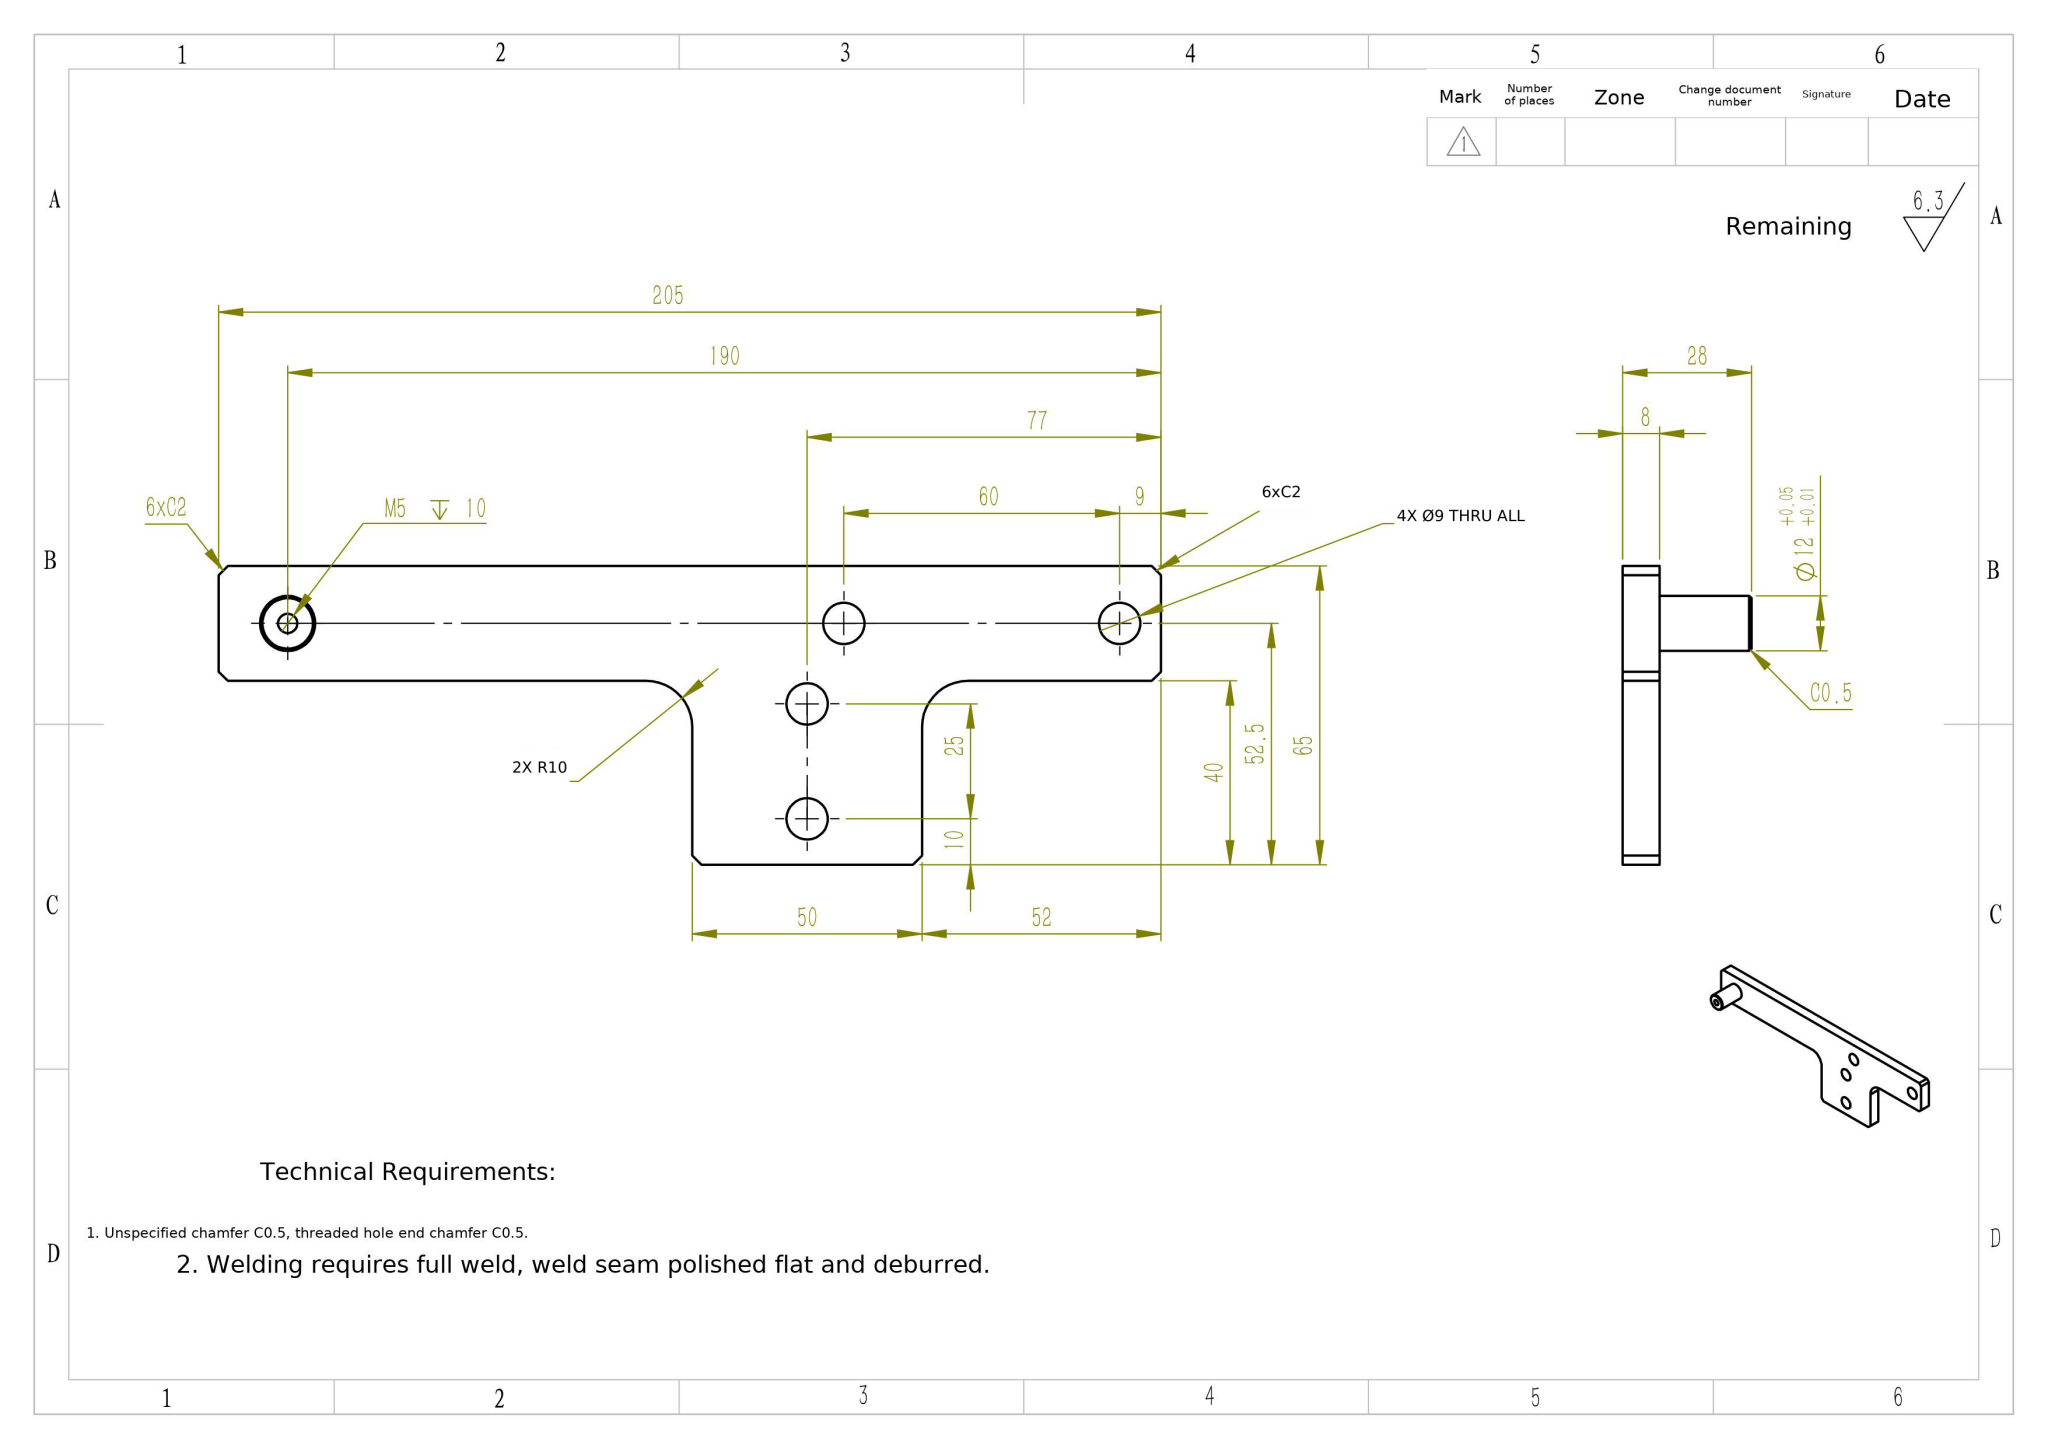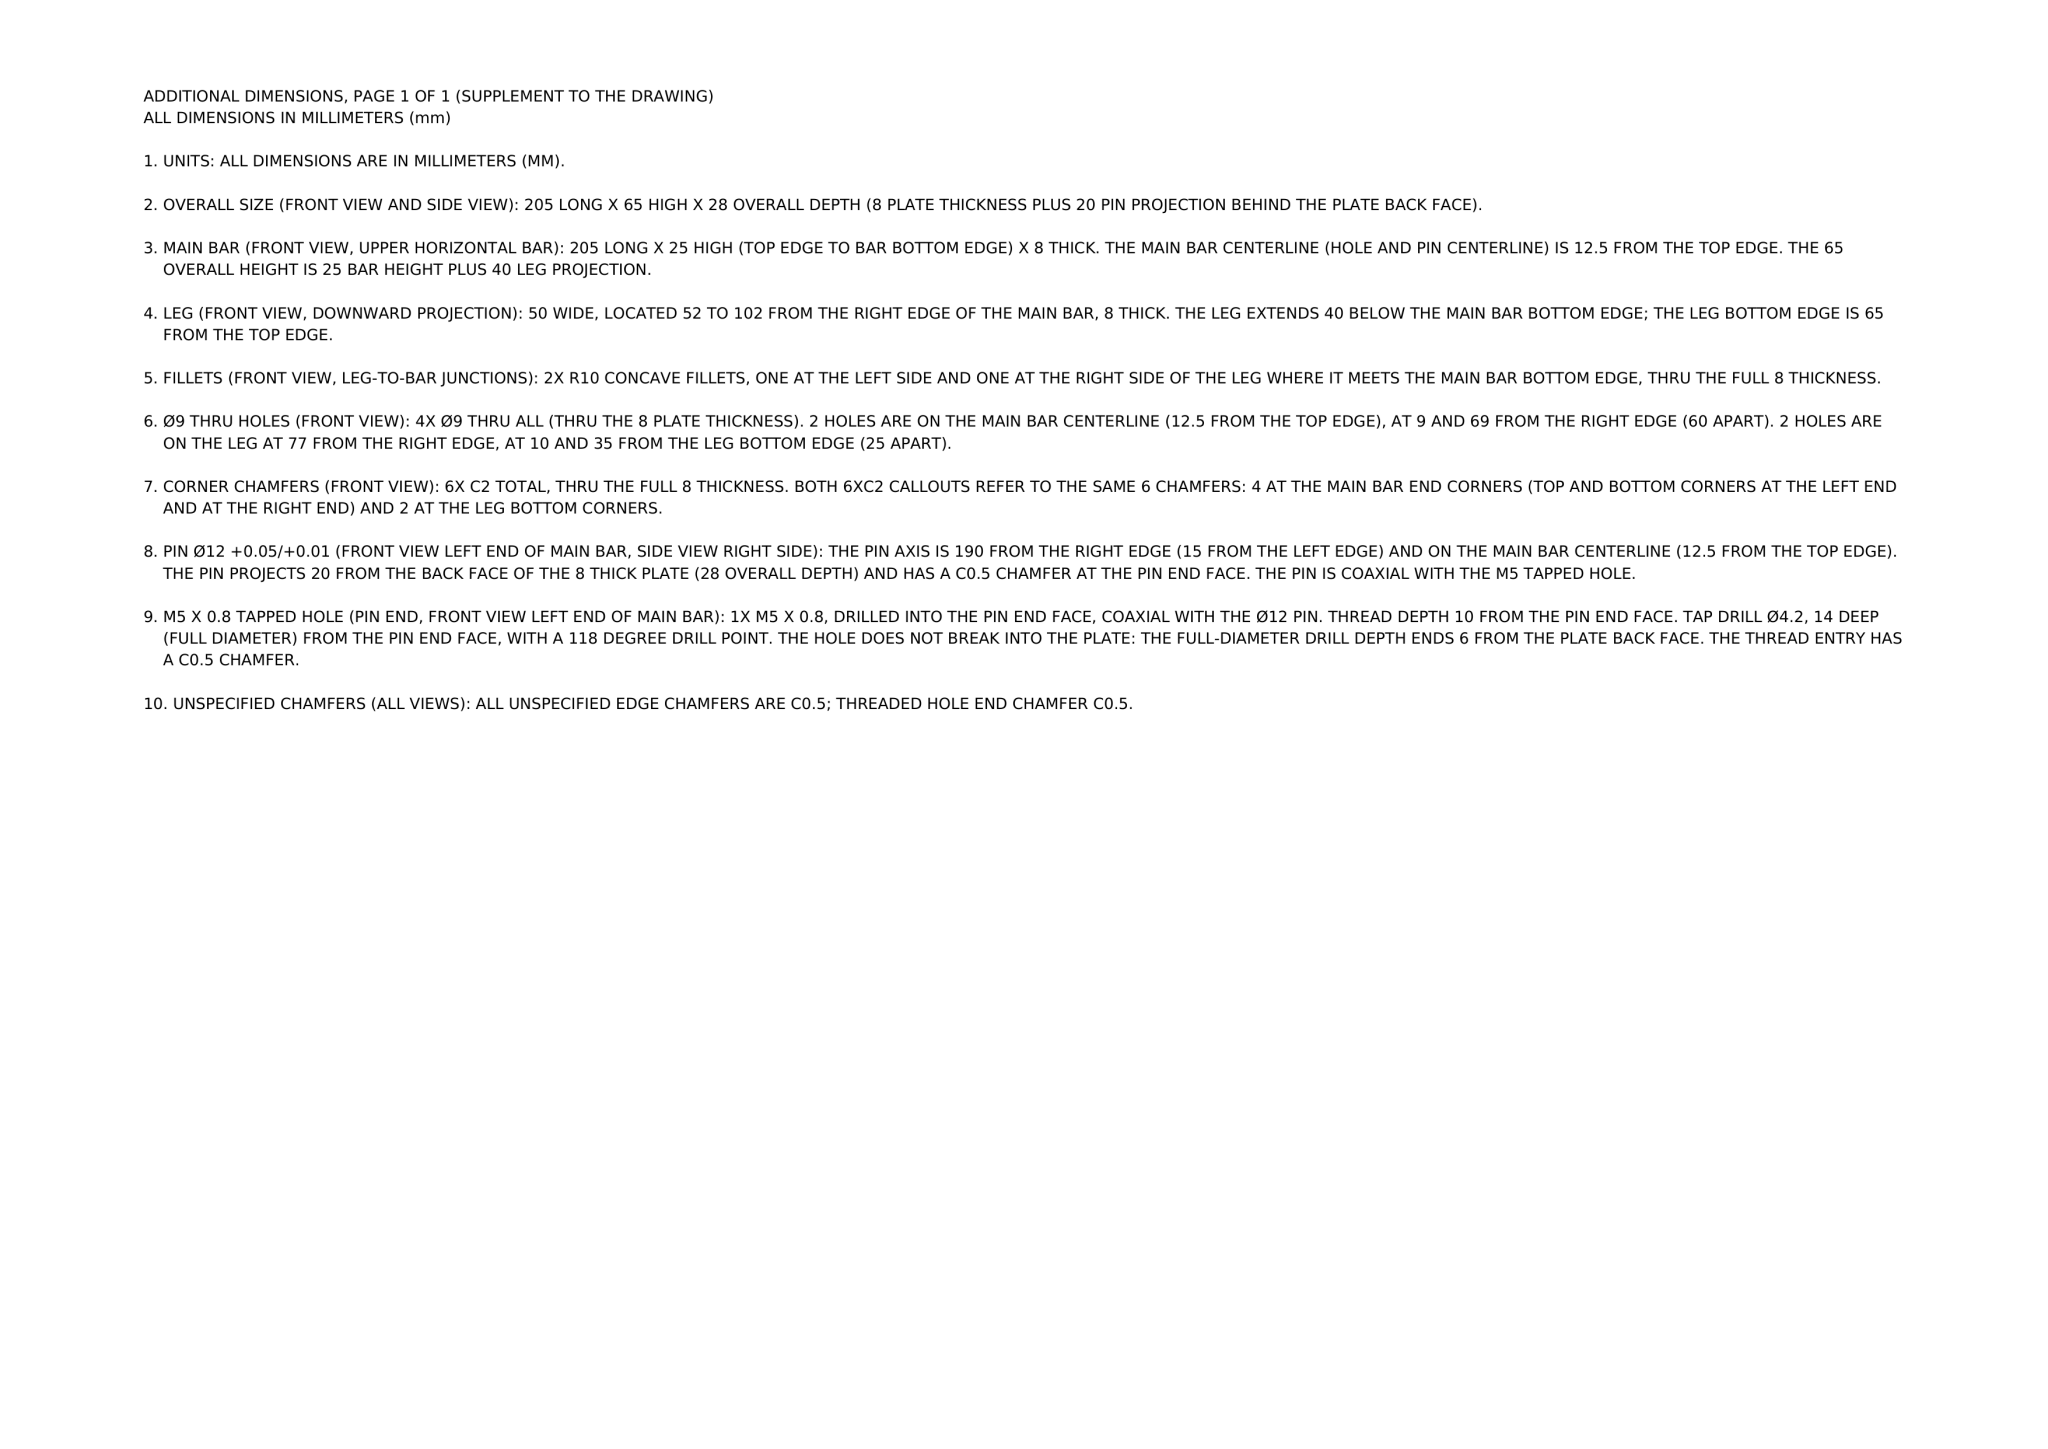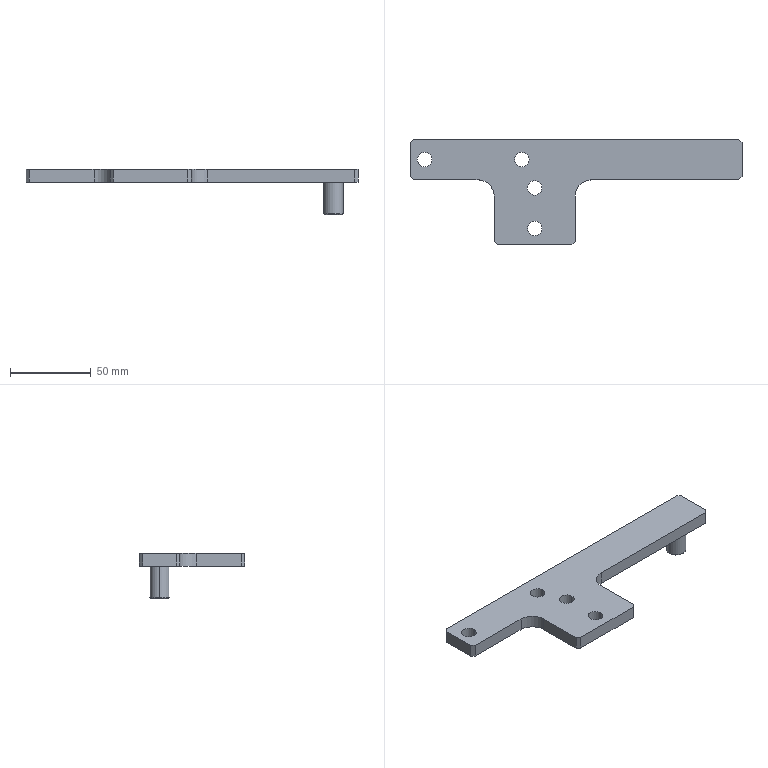Part | NX | mm | 1 solid | 35 faces | box 205 x 65 x 28 mm | volume 57269 mm3 | plane 17 | cylinder 14 | cone 4 | commonest cylinder face diameters 9 x8 4.2 x2 12 x2 20 x2